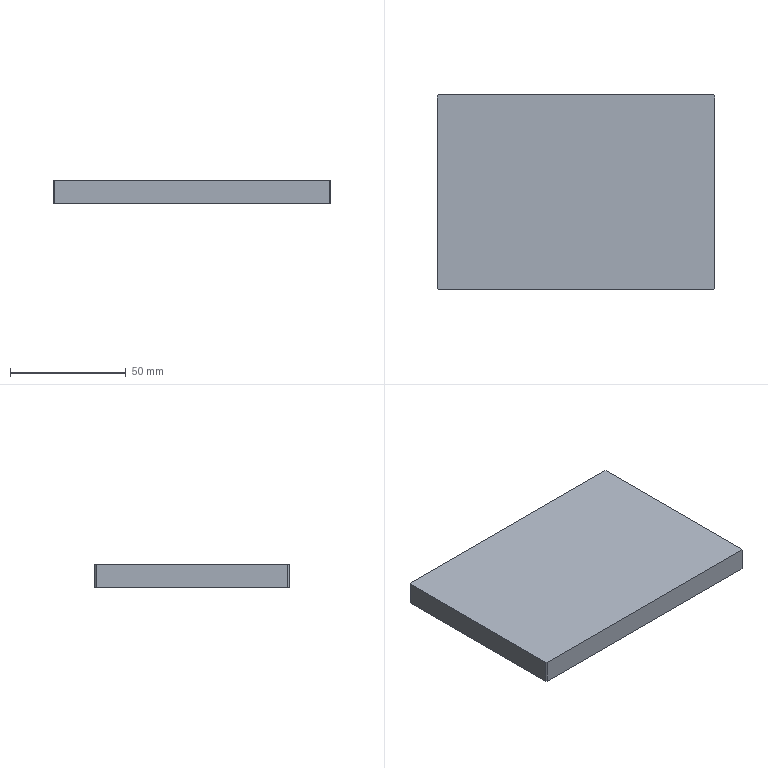Component | SolidWorks | 007-1 | 1 solid | 10 faces | box 120 x 84 x 10 mm | volume 100795 mm3 | plane 10 | material AL6061
build123d program:
from build123d import *

# Parameters (mm, degrees)
SKETCH1_W           = 120
SKETCH1_H           = 84
BOSS_EXTRUDE1_DEPTH = 10
CHAMFER1_SIZE       = 0.5


with BuildPart() as part:
    # Sketch1 → Boss-Extrude1 (new body)
    with BuildSketch(Plane.XY):
        Rectangle(SKETCH1_W, SKETCH1_H)
    extrude(amount=BOSS_EXTRUDE1_DEPTH)

    # Chamfer1
    chamfer1_edges = [part.edges().sort_by_distance(p)[0] for p in [
        (60, -42, 5),
        (-60, -42, 5),
        (-60, 42, 5),
        (60, 42, 5),
    ]]
    chamfer(chamfer1_edges, length=CHAMFER1_SIZE)


solid = part.part

# Placed as in the assembly
solid = solid.moved(Location((-240.455, -63.942, -139.304), (0, 0, 0)))